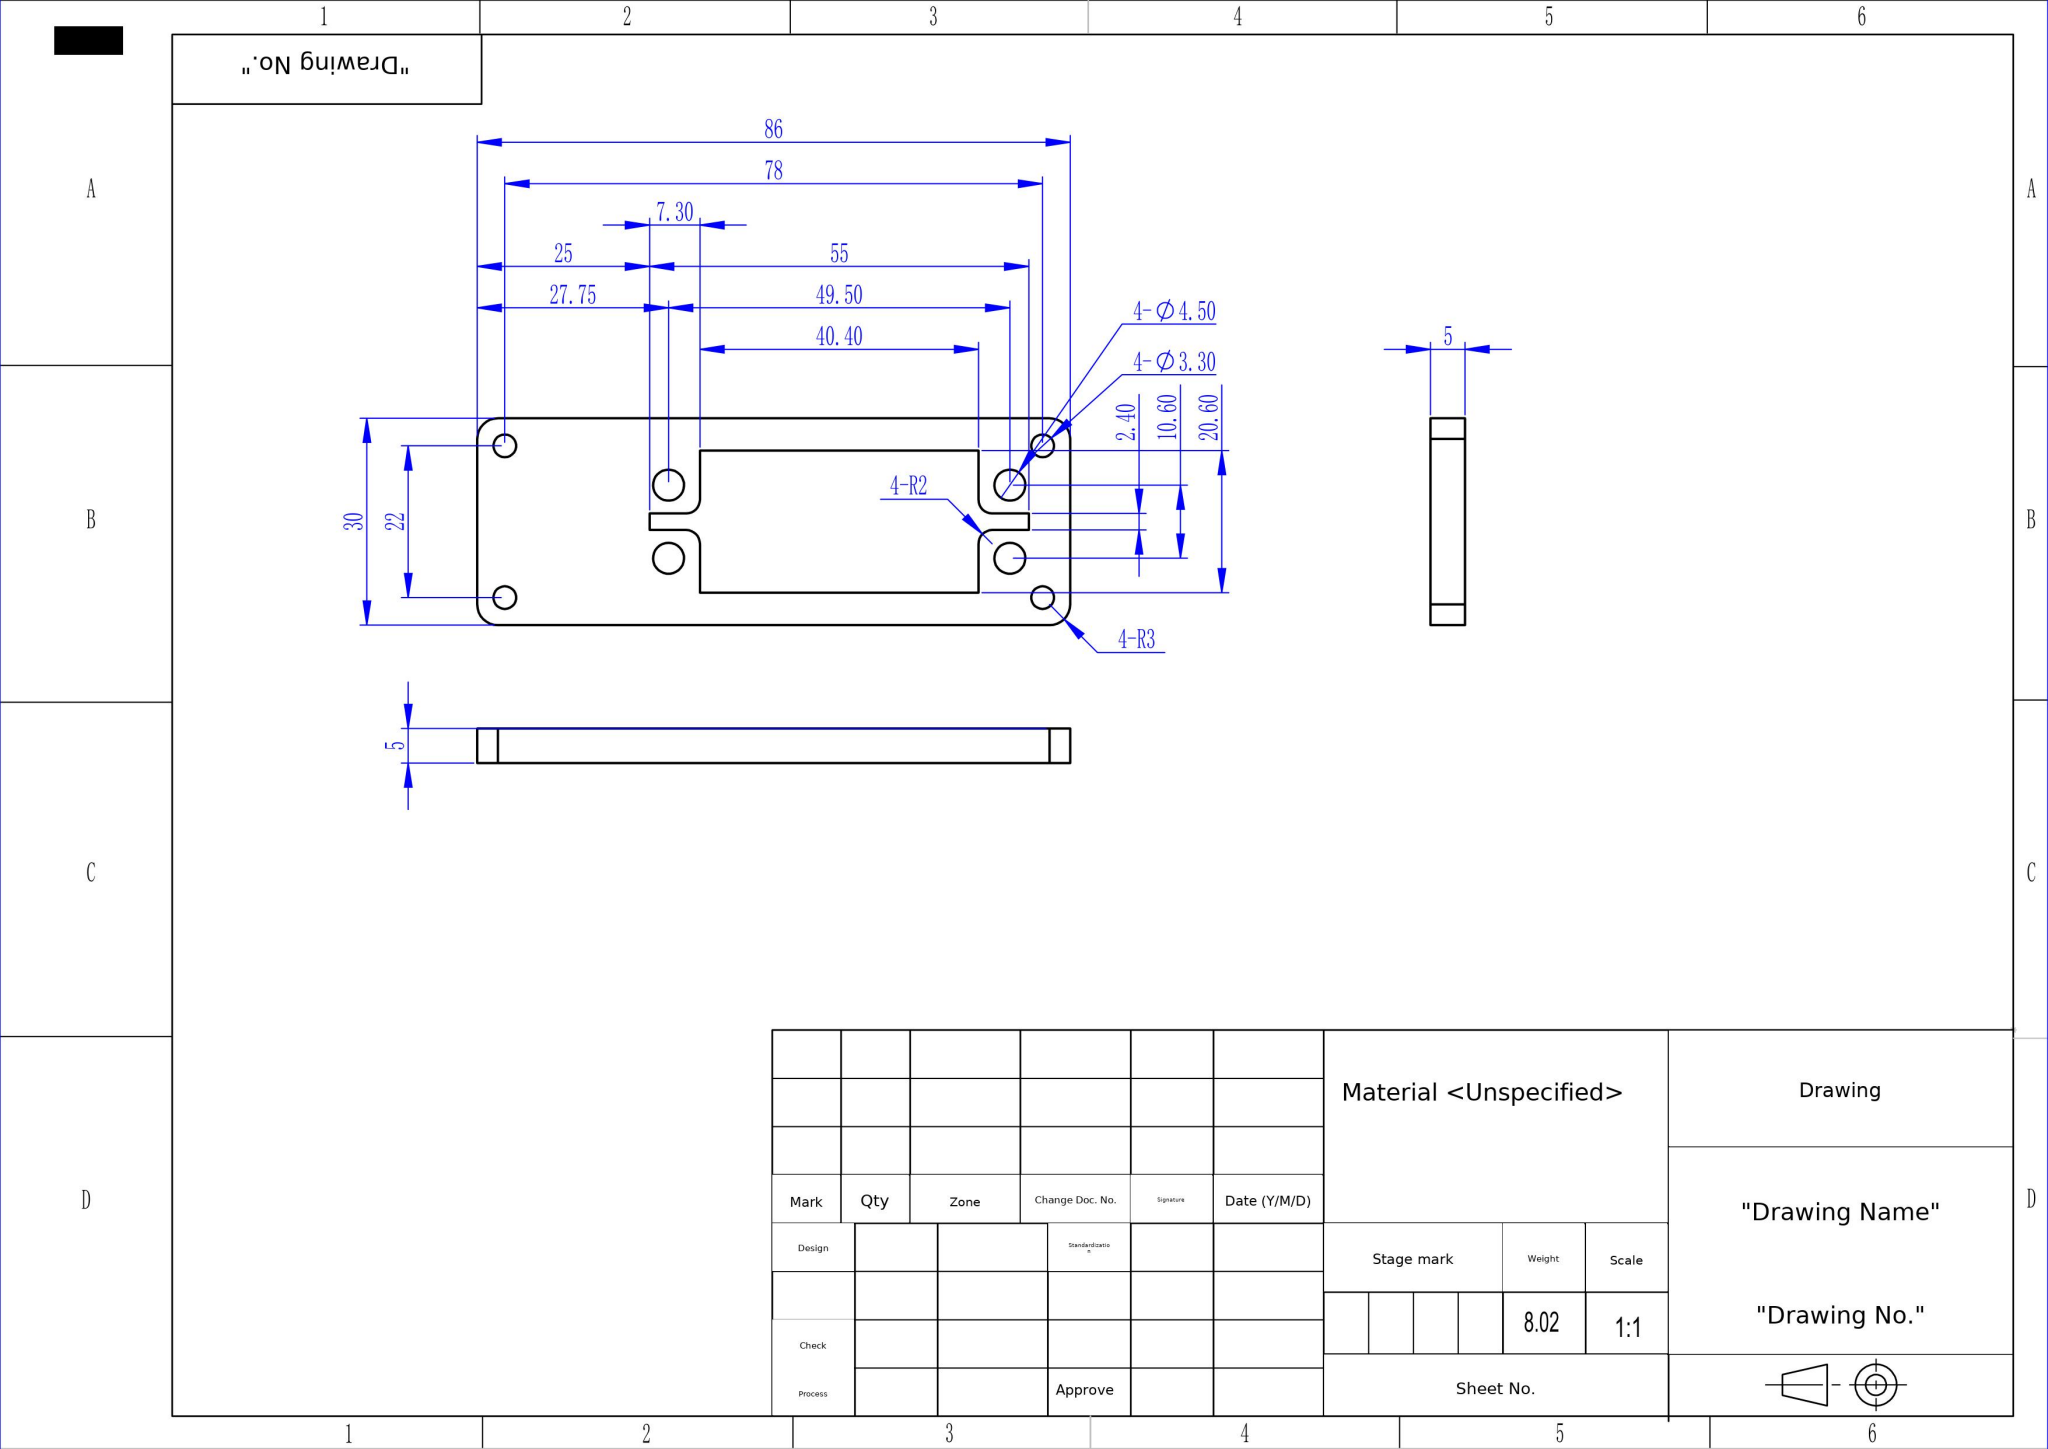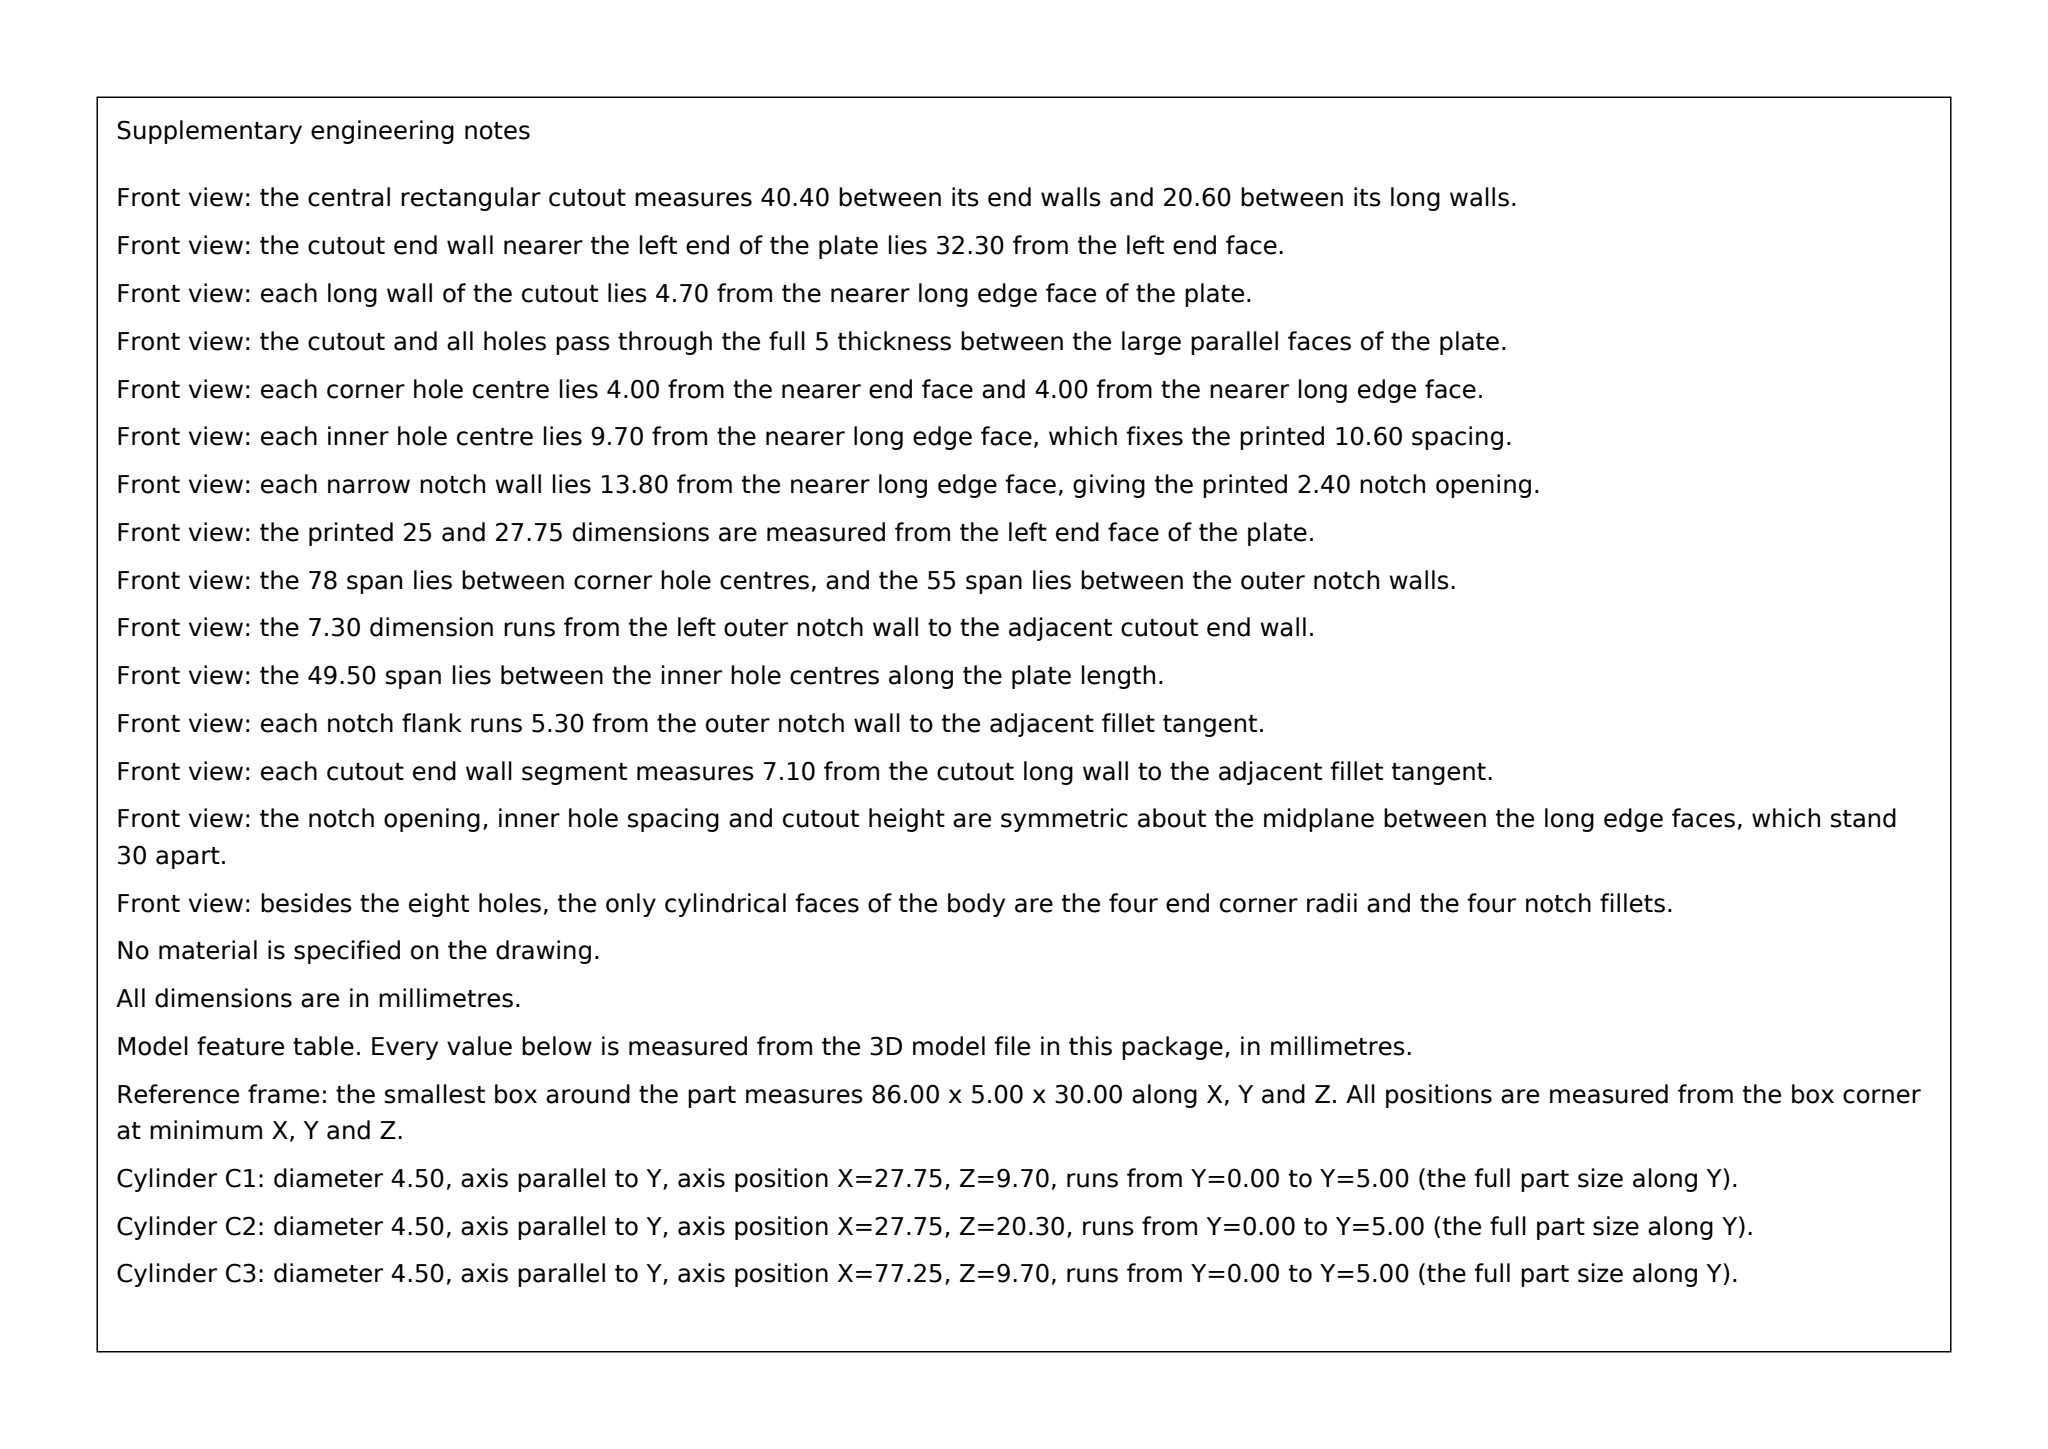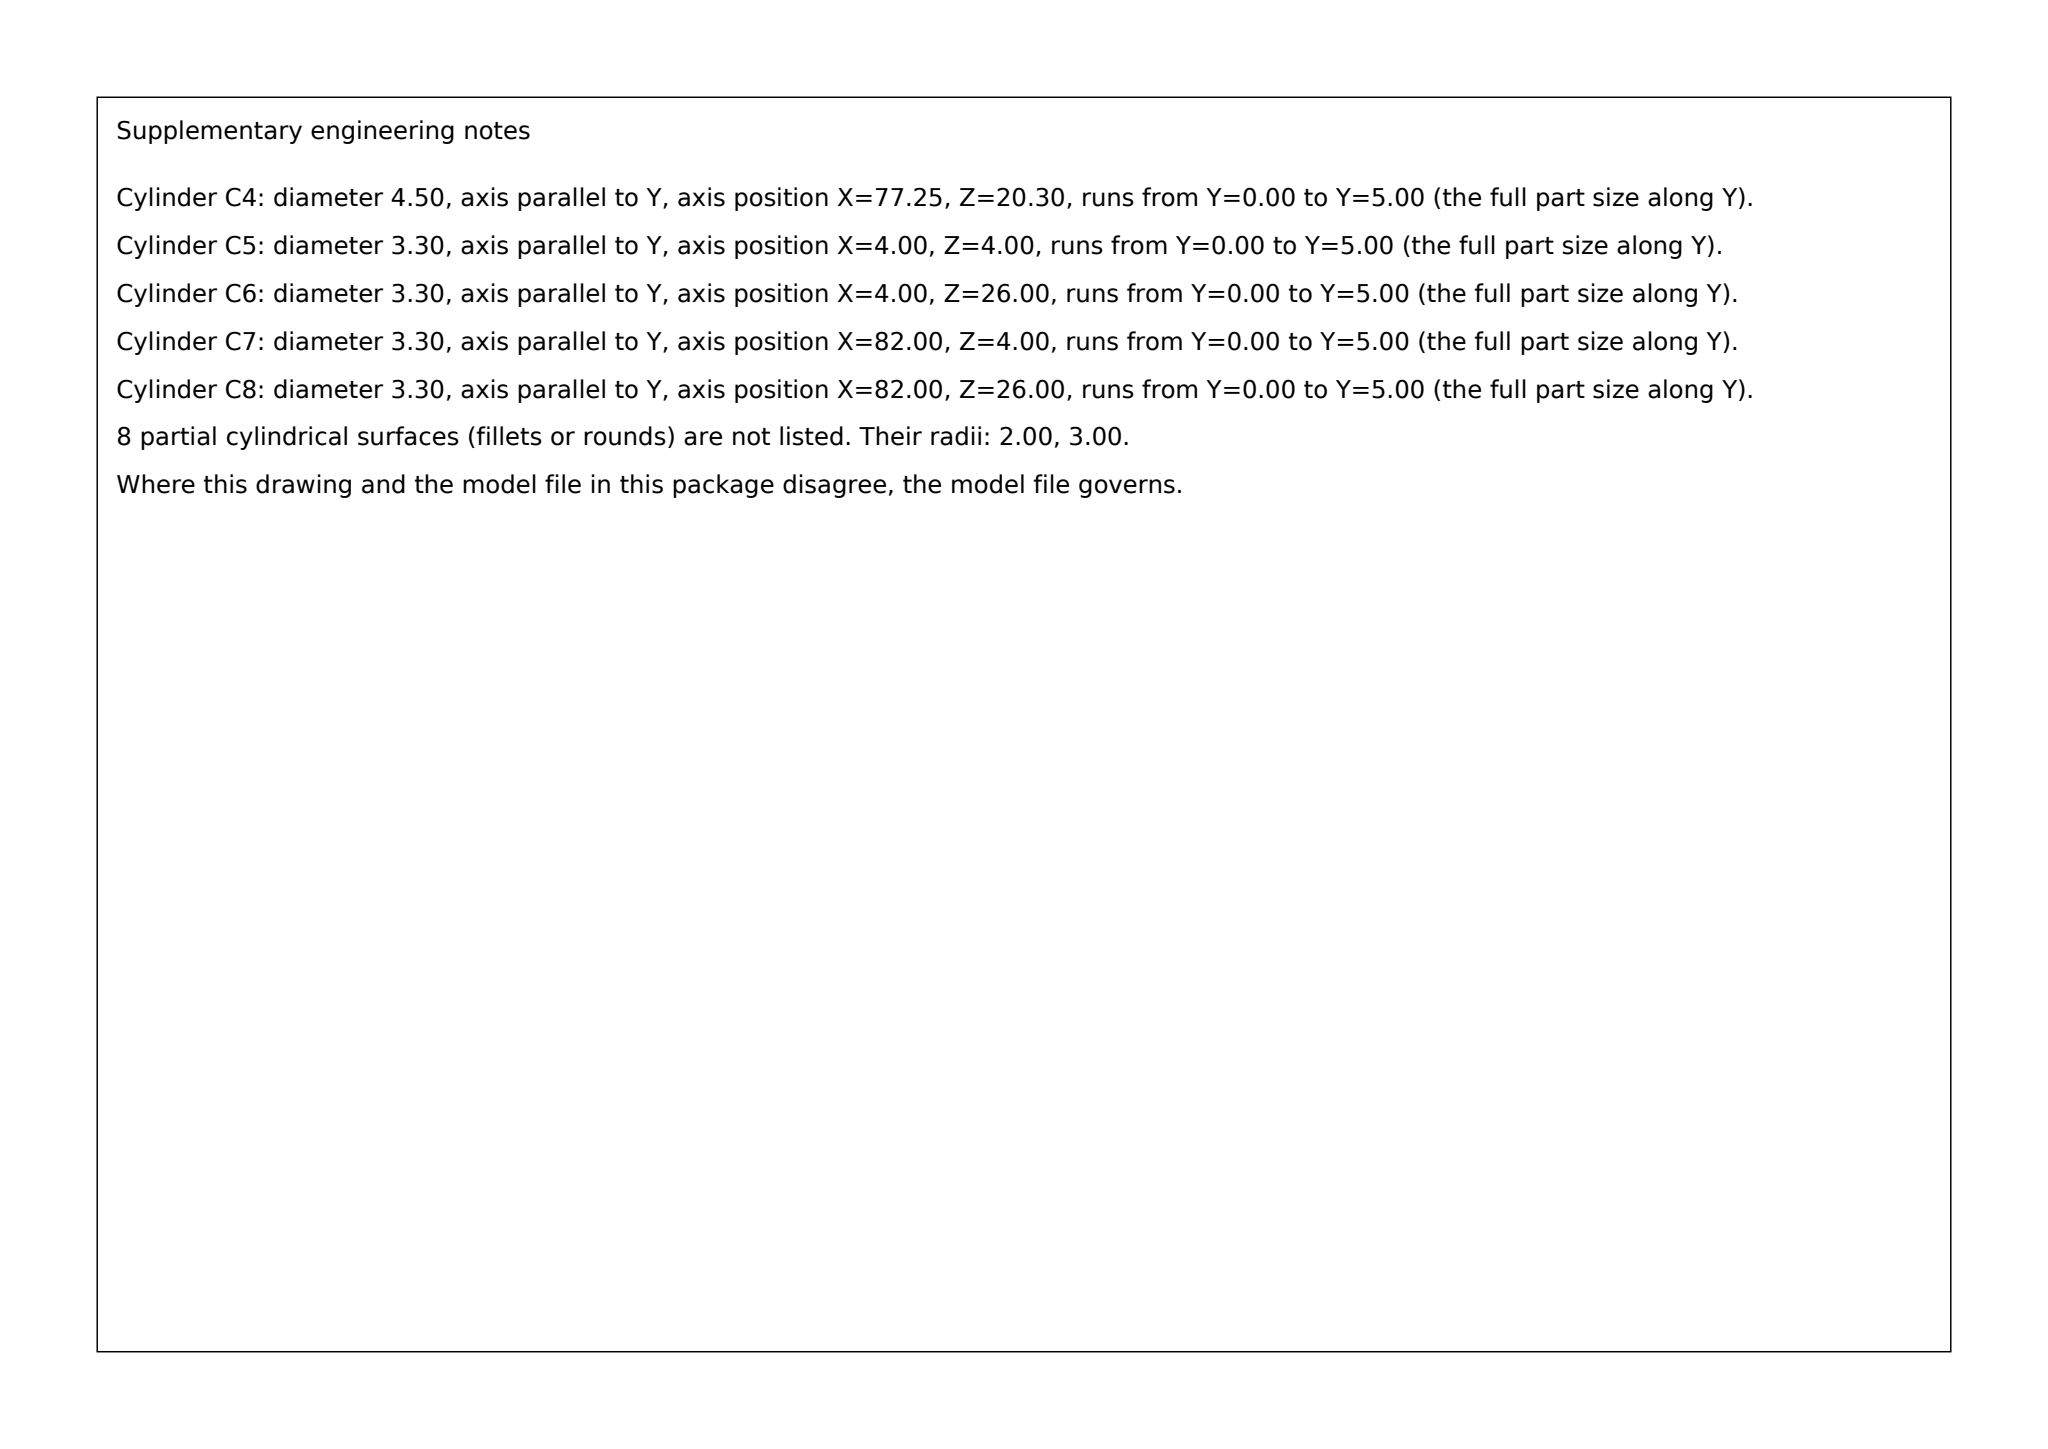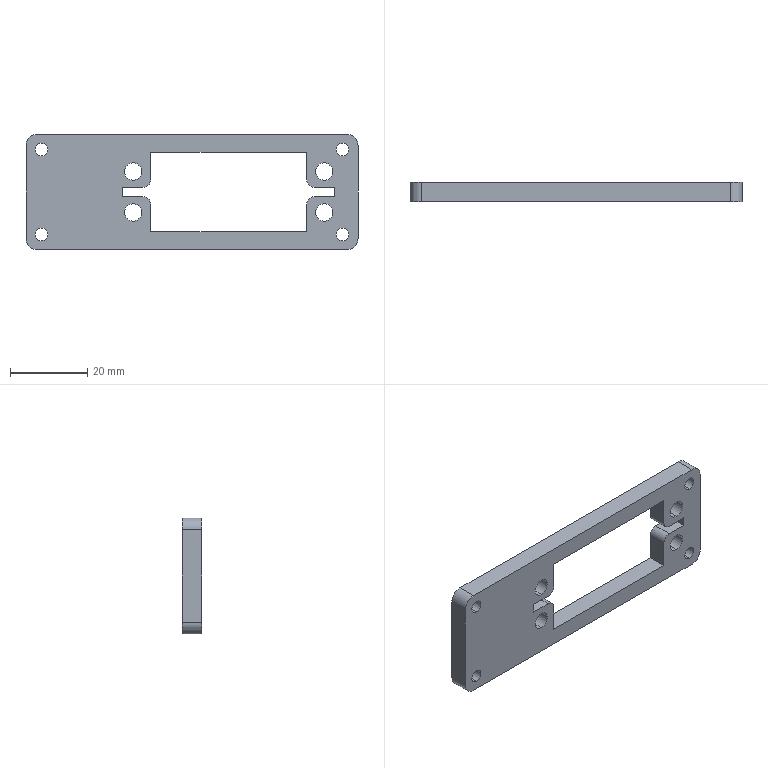Part | SolidWorks | mm | 1 solid | 42 faces | box 86 x 5 x 30 mm | volume 8019 mm3 | cylinder 24 | plane 18 | commonest cylinder face diameters 4.5 x8 3.3 x8 6 x4 4 x4
Drawing notes:
4-Ø4.00 RELIEF HOLES THRU AT SLOT/POCKET JUNCTION | from the solid: cylinders dia 4.0, axis y, length 5.0 (= full 5 thk), qty 4
Ø4.00 RELIEF CTRS: 30.30 & 74.70 FROM LH END, 11.80 & 18.20 FROM BTM | from the solid: 4.0 dia cyl pos (30.3,11.8),(30.3,18.2),(74.7,11.8),(74.7,18.2); bbox 86x30
build123d program:
from build123d import *

# Parameters (mm, degrees)
SKETCH1_R           = 1.65
SKETCH1_R_2         = 2.25
BOSS_EXTRUDE1_DEPTH = 5
FILLET1_R           = 2


with BuildPart() as part:
    # Sketch1 → Boss-Extrude1 (new body)
    with BuildSketch(Plane(origin=(0, 0, 0), x_dir=(1, 0, 0), z_dir=(0, 1, 0))):
        with BuildLine():
            ThreePointArc((43, 12), (42.121, 14.121), (40, 15))
            Line((40, 15), (-40, 15))
            ThreePointArc((-40, 15), (-42.121, 14.121), (-43, 12))
            Line((-43, 12), (-43, -12))
            ThreePointArc((-43, -12), (-42.121, -14.121), (-40, -15))
            Line((-40, -15), (40, -15))
            ThreePointArc((40, -15), (42.121, -14.121), (43, -12))
            Line((43, -12), (43, 12))
        make_face()
        with Locations(Location((-39, 11, 0), (0, 0, 270))):
            Circle(SKETCH1_R, mode=Mode.SUBTRACT)
        with Locations(Location((-39, -11, 0), (0, 0, 270))):
            Circle(SKETCH1_R, mode=Mode.SUBTRACT)
        with Locations(Location((39, -11, 0), (0, 0, 270))):
            Circle(SKETCH1_R, mode=Mode.SUBTRACT)
        with Locations(Location((39, 11, 0), (0, 0, 270))):
            Circle(SKETCH1_R, mode=Mode.SUBTRACT)
        Polygon((-18, -1.2), (-18, 1.2), (-10.7, 1.2), (-10.7, 10.3), (29.7, 10.3), (29.7, 1.2), (37, 1.2), (37, -1.2), (29.7, -1.2), (29.7, -10.3), (-10.7, -10.3), (-10.7, -1.2), align=None, mode=Mode.SUBTRACT)
        with Locations(Location((-15.25, 5.3, 0), (0, 0, 270))):
            Circle(SKETCH1_R_2, mode=Mode.SUBTRACT)
        with Locations(Location((-15.25, -5.3, 0), (0, 0, 270))):
            Circle(SKETCH1_R_2, mode=Mode.SUBTRACT)
        with Locations(Location((34.25, 5.3, 0), (0, 0, 270))):
            Circle(SKETCH1_R_2, mode=Mode.SUBTRACT)
        with Locations(Location((34.25, -5.3, 0), (0, 0, 270))):
            Circle(SKETCH1_R_2, mode=Mode.SUBTRACT)
    extrude(amount=BOSS_EXTRUDE1_DEPTH)

    # Fillet1
    fillet1_edges = [part.edges().sort_by_distance(p)[0] for p in [
        (-10.7, 2.5, 1.2),
        (29.7, 2.5, 1.2),
        (29.7, 2.5, -1.2),
        (-10.7, 2.5, -1.2),
    ]]
    fillet(fillet1_edges, radius=FILLET1_R)


solid = part.part